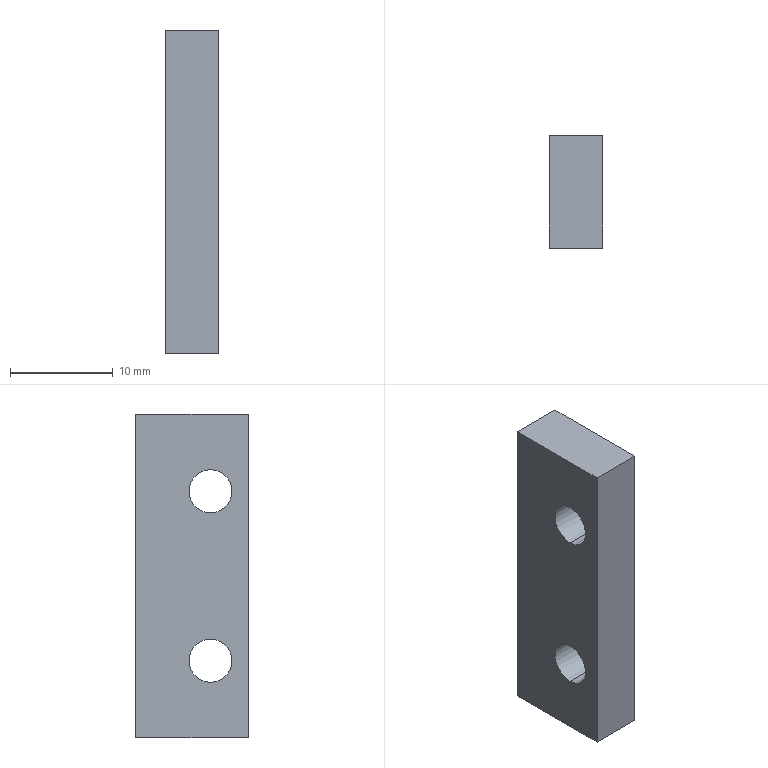Component | SolidWorks | PointedHeadBaseInsert-2 | 1 solid | 10 faces | box 5.2 x 11 x 31.5 mm | volume 1658 mm3 | plane 6 | cylinder 4 | commonest cylinder face diameters 4.2 x4
build123d program:
from build123d import *

# Parameters (mm, degrees)
SKETCH1_W             = 5.2
SKETCH1_H             = 31.5
EXTRUDE1_DEPTH        = 11
M5_TAPPED_HOLE1_D     = 4.2
M5_TAPPED_HOLE1_DEPTH = 14
M5_TAPPED_HOLE1_TIP   = 1.262


with BuildPart() as part:
    # Sketch1 → Extrude1 (new body)
    with BuildSketch(Plane(origin=(0, 0, 0), x_dir=(1, 0, 0), z_dir=(0, 1, 0))):
        with Locations((2.6, -15.75)):
            Rectangle(SKETCH1_W, SKETCH1_H)
    extrude(amount=EXTRUDE1_DEPTH)

    # M5 Tapped Hole1
    with Locations(Plane.ZY):
        with Locations((7.5, 3.7), (24, 3.7)):
            Hole(M5_TAPPED_HOLE1_D / 2, depth=M5_TAPPED_HOLE1_DEPTH)
            with Locations((0, 0, -(M5_TAPPED_HOLE1_DEPTH + M5_TAPPED_HOLE1_TIP / 2))):  # 118° drill point
                Cone(0, M5_TAPPED_HOLE1_D / 2, M5_TAPPED_HOLE1_TIP, mode=Mode.SUBTRACT)


solid = part.part

# Placed as in the assembly
solid = solid.moved(Location((19.917, 66.172, -70.887), (0, 0, 0)))
STEP:
#1=COLOUR_RGB('',0.7922,0.8196,0.9333);
#2=FILL_AREA_STYLE_COLOUR('',#1);
#3=FILL_AREA_STYLE('',(#2));
#4=SURFACE_STYLE_FILL_AREA(#3);
#5=SURFACE_SIDE_STYLE('',(#4));
#6=SURFACE_STYLE_USAGE(.BOTH.,#5);
#7=PRESENTATION_STYLE_ASSIGNMENT((#6));
#8=CARTESIAN_POINT('',(0.9889,2.751,-2.578));
#9=VERTEX_POINT('',#8);
#10=CARTESIAN_POINT('',(0.9889,2.751,-2.413));
#11=VERTEX_POINT('',#10);
#12=CARTESIAN_POINT('',(0.9889,2.751,-2.496));
#13=DIRECTION('',(-1.,0.,0.));
#14=DIRECTION('',(0.,0.,1.));
#15=AXIS2_PLACEMENT_3D('',#12,#13,#14);
#16=CIRCLE('',#15,0.08268);
#17=EDGE_CURVE('',#9,#11,#16,.T.);
#18=ORIENTED_EDGE('',*,*,#17,.F.);
#19=CARTESIAN_POINT('',(0.7841,2.751,-2.578));
#20=VERTEX_POINT('',#19);
#21=CARTESIAN_POINT('',(0.7841,2.751,-2.578));
#22=DIRECTION('',(-1.,0.,0.));
#23=VECTOR('',#22,39.37);
#24=LINE('',#21,#23);
#25=EDGE_CURVE('',#9,#20,#24,.T.);
#26=ORIENTED_EDGE('',*,*,#25,.T.);
#27=CARTESIAN_POINT('',(0.7841,2.751,-2.413));
#28=VERTEX_POINT('',#27);
#29=CARTESIAN_POINT('',(0.7841,2.751,-2.496));
#30=DIRECTION('',(-1.,0.,0.));
#31=DIRECTION('',(0.,0.,1.));
#32=AXIS2_PLACEMENT_3D('',#29,#30,#31);
#33=CIRCLE('',#32,0.08268);
#34=EDGE_CURVE('',#20,#28,#33,.T.);
#35=ORIENTED_EDGE('',*,*,#34,.T.);
#36=CARTESIAN_POINT('',(0.7841,2.751,-2.413));
#37=DIRECTION('',(-1.,0.,0.));
#38=VECTOR('',#37,39.37);
#39=LINE('',#36,#38);
#40=EDGE_CURVE('',#11,#28,#39,.T.);
#41=ORIENTED_EDGE('',*,*,#40,.F.);
#42=EDGE_LOOP('',(#18,#26,#35,#41));
#43=FACE_OUTER_BOUND('',#42,.T.);
#44=CARTESIAN_POINT('',(0.7841,2.751,-2.496));
#45=DIRECTION('',(-1.,0.,0.));
#46=DIRECTION('',(0.,0.,1.));
#47=AXIS2_PLACEMENT_3D('',#44,#45,#46);
#48=CYLINDRICAL_SURFACE('',#47,0.08268);
#49=ADVANCED_FACE('',(#43),#48,.F.);
#50=CARTESIAN_POINT('',(0.9889,2.751,-1.929));
#51=VERTEX_POINT('',#50);
#52=CARTESIAN_POINT('',(0.9889,2.751,-1.763));
#53=VERTEX_POINT('',#52);
#54=CARTESIAN_POINT('',(0.9889,2.751,-1.846));
#55=DIRECTION('',(-1.,0.,0.));
#56=DIRECTION('',(0.,0.,1.));
#57=AXIS2_PLACEMENT_3D('',#54,#55,#56);
#58=CIRCLE('',#57,0.08268);
#59=EDGE_CURVE('',#51,#53,#58,.T.);
#60=ORIENTED_EDGE('',*,*,#59,.F.);
#61=CARTESIAN_POINT('',(0.7841,2.751,-1.929));
#62=VERTEX_POINT('',#61);
#63=CARTESIAN_POINT('',(0.7841,2.751,-1.929));
#64=DIRECTION('',(-1.,0.,0.));
#65=VECTOR('',#64,39.37);
#66=LINE('',#63,#65);
#67=EDGE_CURVE('',#51,#62,#66,.T.);
#68=ORIENTED_EDGE('',*,*,#67,.T.);
#69=CARTESIAN_POINT('',(0.7841,2.751,-1.763));
#70=VERTEX_POINT('',#69);
#71=CARTESIAN_POINT('',(0.7841,2.751,-1.846));
#72=DIRECTION('',(-1.,0.,0.));
#73=DIRECTION('',(0.,0.,1.));
#74=AXIS2_PLACEMENT_3D('',#71,#72,#73);
#75=CIRCLE('',#74,0.08268);
#76=EDGE_CURVE('',#62,#70,#75,.T.);
#77=ORIENTED_EDGE('',*,*,#76,.T.);
#78=CARTESIAN_POINT('',(0.7841,2.751,-1.763));
#79=DIRECTION('',(-1.,0.,0.));
#80=VECTOR('',#79,39.37);
#81=LINE('',#78,#80);
#82=EDGE_CURVE('',#53,#70,#81,.T.);
#83=ORIENTED_EDGE('',*,*,#82,.F.);
#84=EDGE_LOOP('',(#60,#68,#77,#83));
#85=FACE_OUTER_BOUND('',#84,.T.);
#86=CARTESIAN_POINT('',(0.7841,2.751,-1.846));
#87=DIRECTION('',(-1.,0.,0.));
#88=DIRECTION('',(0.,0.,1.));
#89=AXIS2_PLACEMENT_3D('',#86,#87,#88);
#90=CYLINDRICAL_SURFACE('',#89,0.08268);
#91=ADVANCED_FACE('',(#85),#90,.F.);
#92=CARTESIAN_POINT('',(0.7841,2.751,-2.496));
#93=DIRECTION('',(-1.,0.,0.));
#94=DIRECTION('',(0.,0.,1.));
#95=AXIS2_PLACEMENT_3D('',#92,#93,#94);
#96=CIRCLE('',#95,0.08268);
#97=EDGE_CURVE('',#28,#20,#96,.T.);
#98=ORIENTED_EDGE('',*,*,#97,.F.);
#99=ORIENTED_EDGE('',*,*,#34,.F.);
#100=EDGE_LOOP('',(#98,#99));
#101=FACE_BOUND('',#100,.T.);
#102=CARTESIAN_POINT('',(0.7841,2.751,-1.846));
#103=DIRECTION('',(-1.,0.,0.));
#104=DIRECTION('',(0.,0.,1.));
#105=AXIS2_PLACEMENT_3D('',#102,#103,#104);
#106=CIRCLE('',#105,0.08268);
#107=EDGE_CURVE('',#70,#62,#106,.T.);
#108=ORIENTED_EDGE('',*,*,#107,.F.);
#109=ORIENTED_EDGE('',*,*,#76,.F.);
#110=EDGE_LOOP('',(#108,#109));
#111=FACE_BOUND('',#110,.T.);
#112=CARTESIAN_POINT('',(0.7841,2.605,-2.791));
#113=VERTEX_POINT('',#112);
#114=CARTESIAN_POINT('',(0.7841,2.605,-1.551));
#115=VERTEX_POINT('',#114);
#116=CARTESIAN_POINT('',(0.7841,2.605,-2.791));
#117=DIRECTION('',(0.,0.,1.));
#118=VECTOR('',#117,39.37);
#119=LINE('',#116,#118);
#120=EDGE_CURVE('',#113,#115,#119,.T.);
#121=ORIENTED_EDGE('',*,*,#120,.T.);
#122=CARTESIAN_POINT('',(0.7841,3.038,-1.551));
#123=VERTEX_POINT('',#122);
#124=CARTESIAN_POINT('',(0.7841,3.038,-1.551));
#125=DIRECTION('',(0.,-1.,0.));
#126=VECTOR('',#125,39.37);
#127=LINE('',#124,#126);
#128=EDGE_CURVE('',#123,#115,#127,.T.);
#129=ORIENTED_EDGE('',*,*,#128,.F.);
#130=CARTESIAN_POINT('',(0.7841,3.038,-2.791));
#131=VERTEX_POINT('',#130);
#132=CARTESIAN_POINT('',(0.7841,3.038,-2.791));
#133=DIRECTION('',(0.,0.,1.));
#134=VECTOR('',#133,39.37);
#135=LINE('',#132,#134);
#136=EDGE_CURVE('',#131,#123,#135,.T.);
#137=ORIENTED_EDGE('',*,*,#136,.F.);
#138=CARTESIAN_POINT('',(0.7841,3.038,-2.791));
#139=DIRECTION('',(0.,-1.,0.));
#140=VECTOR('',#139,39.37);
#141=LINE('',#138,#140);
#142=EDGE_CURVE('',#131,#113,#141,.T.);
#143=ORIENTED_EDGE('',*,*,#142,.T.);
#144=EDGE_LOOP('',(#121,#129,#137,#143));
#145=FACE_OUTER_BOUND('',#144,.T.);
#146=CARTESIAN_POINT('',(0.7841,3.038,-2.791));
#147=DIRECTION('',(1.,0.,-0.));
#148=DIRECTION('',(-0.,0.,-1.));
#149=AXIS2_PLACEMENT_3D('',#146,#147,#148);
#150=PLANE('',#149);
#151=ADVANCED_FACE('',(#101,#111,#145),#150,.F.);
#152=CARTESIAN_POINT('',(0.9889,2.605,-1.551));
#153=VERTEX_POINT('',#152);
#154=CARTESIAN_POINT('',(0.7841,2.605,-1.551));
#155=DIRECTION('',(1.,0.,0.));
#156=VECTOR('',#155,39.37);
#157=LINE('',#154,#156);
#158=EDGE_CURVE('',#115,#153,#157,.T.);
#159=ORIENTED_EDGE('',*,*,#158,.T.);
#160=CARTESIAN_POINT('',(0.9889,3.038,-1.551));
#161=VERTEX_POINT('',#160);
#162=CARTESIAN_POINT('',(0.9889,3.038,-1.551));
#163=DIRECTION('',(0.,-1.,0.));
#164=VECTOR('',#163,39.37);
#165=LINE('',#162,#164);
#166=EDGE_CURVE('',#161,#153,#165,.T.);
#167=ORIENTED_EDGE('',*,*,#166,.F.);
#168=CARTESIAN_POINT('',(0.7841,3.038,-1.551));
#169=DIRECTION('',(1.,0.,0.));
#170=VECTOR('',#169,39.37);
#171=LINE('',#168,#170);
#172=EDGE_CURVE('',#123,#161,#171,.T.);
#173=ORIENTED_EDGE('',*,*,#172,.F.);
#174=ORIENTED_EDGE('',*,*,#128,.T.);
#175=EDGE_LOOP('',(#159,#167,#173,#174));
#176=FACE_OUTER_BOUND('',#175,.T.);
#177=CARTESIAN_POINT('',(0.7841,3.038,-1.551));
#178=DIRECTION('',(0.,0.,-1.));
#179=DIRECTION('',(-1.,0.,0.));
#180=AXIS2_PLACEMENT_3D('',#177,#178,#179);
#181=PLANE('',#180);
#182=ADVANCED_FACE('',(#176),#181,.F.);
#183=CARTESIAN_POINT('',(0.9889,2.751,-2.496));
#184=DIRECTION('',(-1.,0.,0.));
#185=DIRECTION('',(0.,0.,1.));
#186=AXIS2_PLACEMENT_3D('',#183,#184,#185);
#187=CIRCLE('',#186,0.08268);
#188=EDGE_CURVE('',#11,#9,#187,.T.);
#189=ORIENTED_EDGE('',*,*,#188,.T.);
#190=ORIENTED_EDGE('',*,*,#17,.T.);
#191=EDGE_LOOP('',(#189,#190));
#192=FACE_BOUND('',#191,.T.);
#193=CARTESIAN_POINT('',(0.9889,2.751,-1.846));
#194=DIRECTION('',(-1.,0.,0.));
#195=DIRECTION('',(0.,0.,1.));
#196=AXIS2_PLACEMENT_3D('',#193,#194,#195);
#197=CIRCLE('',#196,0.08268);
#198=EDGE_CURVE('',#53,#51,#197,.T.);
#199=ORIENTED_EDGE('',*,*,#198,.T.);
#200=ORIENTED_EDGE('',*,*,#59,.T.);
#201=EDGE_LOOP('',(#199,#200));
#202=FACE_BOUND('',#201,.T.);
#203=CARTESIAN_POINT('',(0.9889,2.605,-2.791));
#204=VERTEX_POINT('',#203);
#205=CARTESIAN_POINT('',(0.9889,2.605,-2.791));
#206=DIRECTION('',(-0.,0.,-1.));
#207=VECTOR('',#206,39.37);
#208=LINE('',#205,#207);
#209=EDGE_CURVE('',#153,#204,#208,.T.);
#210=ORIENTED_EDGE('',*,*,#209,.T.);
#211=CARTESIAN_POINT('',(0.9889,3.038,-2.791));
#212=VERTEX_POINT('',#211);
#213=CARTESIAN_POINT('',(0.9889,3.038,-2.791));
#214=DIRECTION('',(0.,-1.,0.));
#215=VECTOR('',#214,39.37);
#216=LINE('',#213,#215);
#217=EDGE_CURVE('',#212,#204,#216,.T.);
#218=ORIENTED_EDGE('',*,*,#217,.F.);
#219=CARTESIAN_POINT('',(0.9889,3.038,-2.791));
#220=DIRECTION('',(-0.,0.,-1.));
#221=VECTOR('',#220,39.37);
#222=LINE('',#219,#221);
#223=EDGE_CURVE('',#161,#212,#222,.T.);
#224=ORIENTED_EDGE('',*,*,#223,.F.);
#225=ORIENTED_EDGE('',*,*,#166,.T.);
#226=EDGE_LOOP('',(#210,#218,#224,#225));
#227=FACE_OUTER_BOUND('',#226,.T.);
#228=CARTESIAN_POINT('',(0.9889,3.038,-2.791));
#229=DIRECTION('',(-1.,0.,0.));
#230=DIRECTION('',(0.,0.,1.));
#231=AXIS2_PLACEMENT_3D('',#228,#229,#230);
#232=PLANE('',#231);
#233=ADVANCED_FACE('',(#192,#202,#227),#232,.F.);
#234=CARTESIAN_POINT('',(0.7841,2.605,-2.791));
#235=DIRECTION('',(-1.,0.,0.));
#236=VECTOR('',#235,39.37);
#237=LINE('',#234,#236);
#238=EDGE_CURVE('',#204,#113,#237,.T.);
#239=ORIENTED_EDGE('',*,*,#238,.T.);
#240=ORIENTED_EDGE('',*,*,#142,.F.);
#241=CARTESIAN_POINT('',(0.7841,3.038,-2.791));
#242=DIRECTION('',(-1.,0.,0.));
#243=VECTOR('',#242,39.37);
#244=LINE('',#241,#243);
#245=EDGE_CURVE('',#212,#131,#244,.T.);
#246=ORIENTED_EDGE('',*,*,#245,.F.);
#247=ORIENTED_EDGE('',*,*,#217,.T.);
#248=EDGE_LOOP('',(#239,#240,#246,#247));
#249=FACE_OUTER_BOUND('',#248,.T.);
#250=CARTESIAN_POINT('',(0.7841,3.038,-2.791));
#251=DIRECTION('',(0.,0.,1.));
#252=DIRECTION('',(1.,0.,0.));
#253=AXIS2_PLACEMENT_3D('',#250,#251,#252);
#254=PLANE('',#253);
#255=ADVANCED_FACE('',(#249),#254,.F.);
#256=ORIENTED_EDGE('',*,*,#136,.T.);
#257=ORIENTED_EDGE('',*,*,#172,.T.);
#258=ORIENTED_EDGE('',*,*,#223,.T.);
#259=ORIENTED_EDGE('',*,*,#245,.T.);
#260=EDGE_LOOP('',(#256,#257,#258,#259));
#261=FACE_OUTER_BOUND('',#260,.T.);
#262=CARTESIAN_POINT('',(0.7841,3.038,-1.551));
#263=DIRECTION('',(0.,1.,0.));
#264=DIRECTION('',(0.,0.,1.));
#265=AXIS2_PLACEMENT_3D('',#262,#263,#264);
#266=PLANE('',#265);
#267=ADVANCED_FACE('',(#261),#266,.T.);
#268=ORIENTED_EDGE('',*,*,#120,.F.);
#269=ORIENTED_EDGE('',*,*,#238,.F.);
#270=ORIENTED_EDGE('',*,*,#209,.F.);
#271=ORIENTED_EDGE('',*,*,#158,.F.);
#272=EDGE_LOOP('',(#268,#269,#270,#271));
#273=FACE_OUTER_BOUND('',#272,.T.);
#274=CARTESIAN_POINT('',(0.7841,2.605,-1.551));
#275=DIRECTION('',(0.,1.,0.));
#276=DIRECTION('',(0.,0.,1.));
#277=AXIS2_PLACEMENT_3D('',#274,#275,#276);
#278=PLANE('',#277);
#279=ADVANCED_FACE('',(#273),#278,.F.);
#280=ORIENTED_EDGE('',*,*,#67,.F.);
#281=ORIENTED_EDGE('',*,*,#198,.F.);
#282=ORIENTED_EDGE('',*,*,#82,.T.);
#283=ORIENTED_EDGE('',*,*,#107,.T.);
#284=EDGE_LOOP('',(#280,#281,#282,#283));
#285=FACE_OUTER_BOUND('',#284,.T.);
#286=CARTESIAN_POINT('',(0.7841,2.751,-1.846));
#287=DIRECTION('',(-1.,0.,0.));
#288=DIRECTION('',(0.,0.,1.));
#289=AXIS2_PLACEMENT_3D('',#286,#287,#288);
#290=CYLINDRICAL_SURFACE('',#289,0.08268);
#291=ADVANCED_FACE('',(#285),#290,.F.);
#292=ORIENTED_EDGE('',*,*,#25,.F.);
#293=ORIENTED_EDGE('',*,*,#188,.F.);
#294=ORIENTED_EDGE('',*,*,#40,.T.);
#295=ORIENTED_EDGE('',*,*,#97,.T.);
#296=EDGE_LOOP('',(#292,#293,#294,#295));
#297=FACE_OUTER_BOUND('',#296,.T.);
#298=CARTESIAN_POINT('',(0.7841,2.751,-2.496));
#299=DIRECTION('',(-1.,0.,0.));
#300=DIRECTION('',(0.,0.,1.));
#301=AXIS2_PLACEMENT_3D('',#298,#299,#300);
#302=CYLINDRICAL_SURFACE('',#301,0.08268);
#303=ADVANCED_FACE('',(#297),#302,.F.);
#304=CLOSED_SHELL('',(#49,#91,#151,#182,#233,#255,#267,#279,#291,#303));
#305=MANIFOLD_SOLID_BREP('',#304);
#306=STYLED_ITEM('',(#7),#305);
#307=(LENGTH_UNIT()NAMED_UNIT(*)SI_UNIT($,.METRE.));
#308=LENGTH_MEASURE_WITH_UNIT(LENGTH_MEASURE(0.0254),#307);
#309=DIMENSIONAL_EXPONENTS(1.,0.,0.,0.,0.,0.,0.);
#310=(CONVERSION_BASED_UNIT('',#308)LENGTH_UNIT()NAMED_UNIT(#309));
#311=UNCERTAINTY_MEASURE_WITH_UNIT(LENGTH_MEASURE(0.00001),#310,'','');
#312=(NAMED_UNIT(*)PLANE_ANGLE_UNIT()SI_UNIT($,.RADIAN.));
#313=(NAMED_UNIT(*)SI_UNIT($,.STERADIAN.)SOLID_ANGLE_UNIT());
#314=(GEOMETRIC_REPRESENTATION_CONTEXT(3)GLOBAL_UNCERTAINTY_ASSIGNED_CONTEXT((#311))GLOBAL_UNIT_ASSIGNED_CONTEXT((#310,#312,#313))REPRESENTATION_CONTEXT('',''));
#315=MECHANICAL_DESIGN_GEOMETRIC_PRESENTATION_REPRESENTATION('',(#306),#314);
#316=CARTESIAN_POINT('',(0.,0.,0.));
#317=DIRECTION('',(0.,0.,1.));
#318=DIRECTION('',(1.,0.,0.));
#319=AXIS2_PLACEMENT_3D('',#316,#317,#318);
#320=(LENGTH_UNIT()NAMED_UNIT(*)SI_UNIT($,.METRE.));
#321=LENGTH_MEASURE_WITH_UNIT(LENGTH_MEASURE(0.0254),#320);
#322=DIMENSIONAL_EXPONENTS(1.,0.,0.,0.,0.,0.,0.);
#323=(CONVERSION_BASED_UNIT('',#321)LENGTH_UNIT()NAMED_UNIT(#322));
#324=UNCERTAINTY_MEASURE_WITH_UNIT(LENGTH_MEASURE(0.00001),#323,'','');
#325=(NAMED_UNIT(*)PLANE_ANGLE_UNIT()SI_UNIT($,.RADIAN.));
#326=(NAMED_UNIT(*)SI_UNIT($,.STERADIAN.)SOLID_ANGLE_UNIT());
#327=(GEOMETRIC_REPRESENTATION_CONTEXT(3)GLOBAL_UNCERTAINTY_ASSIGNED_CONTEXT((#324))GLOBAL_UNIT_ASSIGNED_CONTEXT((#323,#325,#326))REPRESENTATION_CONTEXT('',''));
#328=ADVANCED_BREP_SHAPE_REPRESENTATION('',(#305,#319),#327);
#329=PRESENTATION_LAYER_ASSIGNMENT('','',(#306));